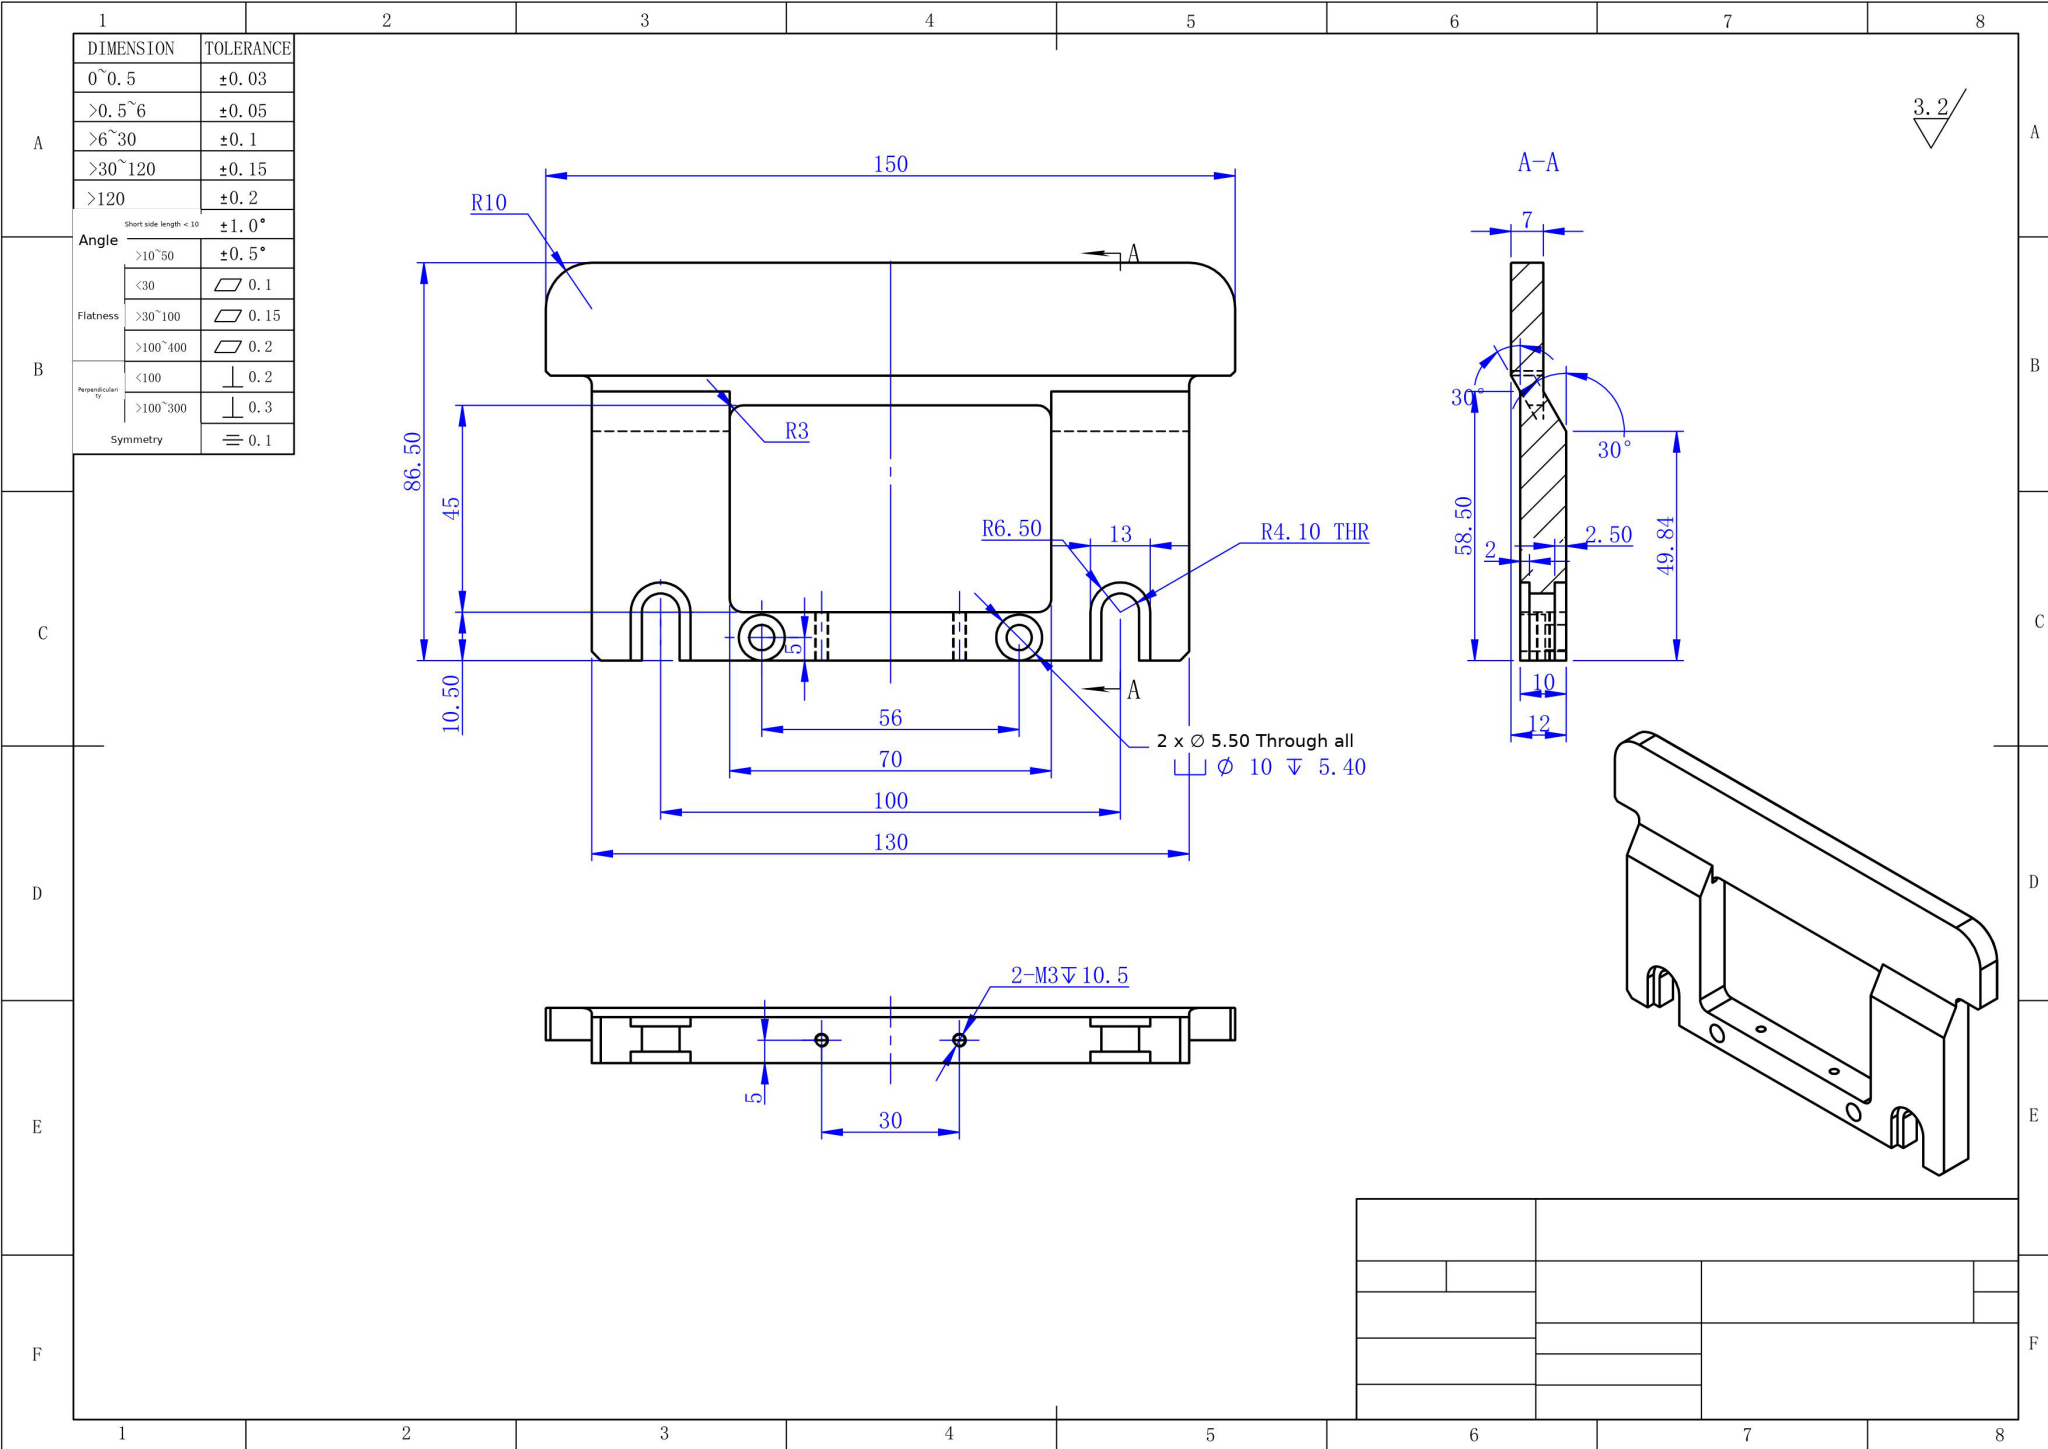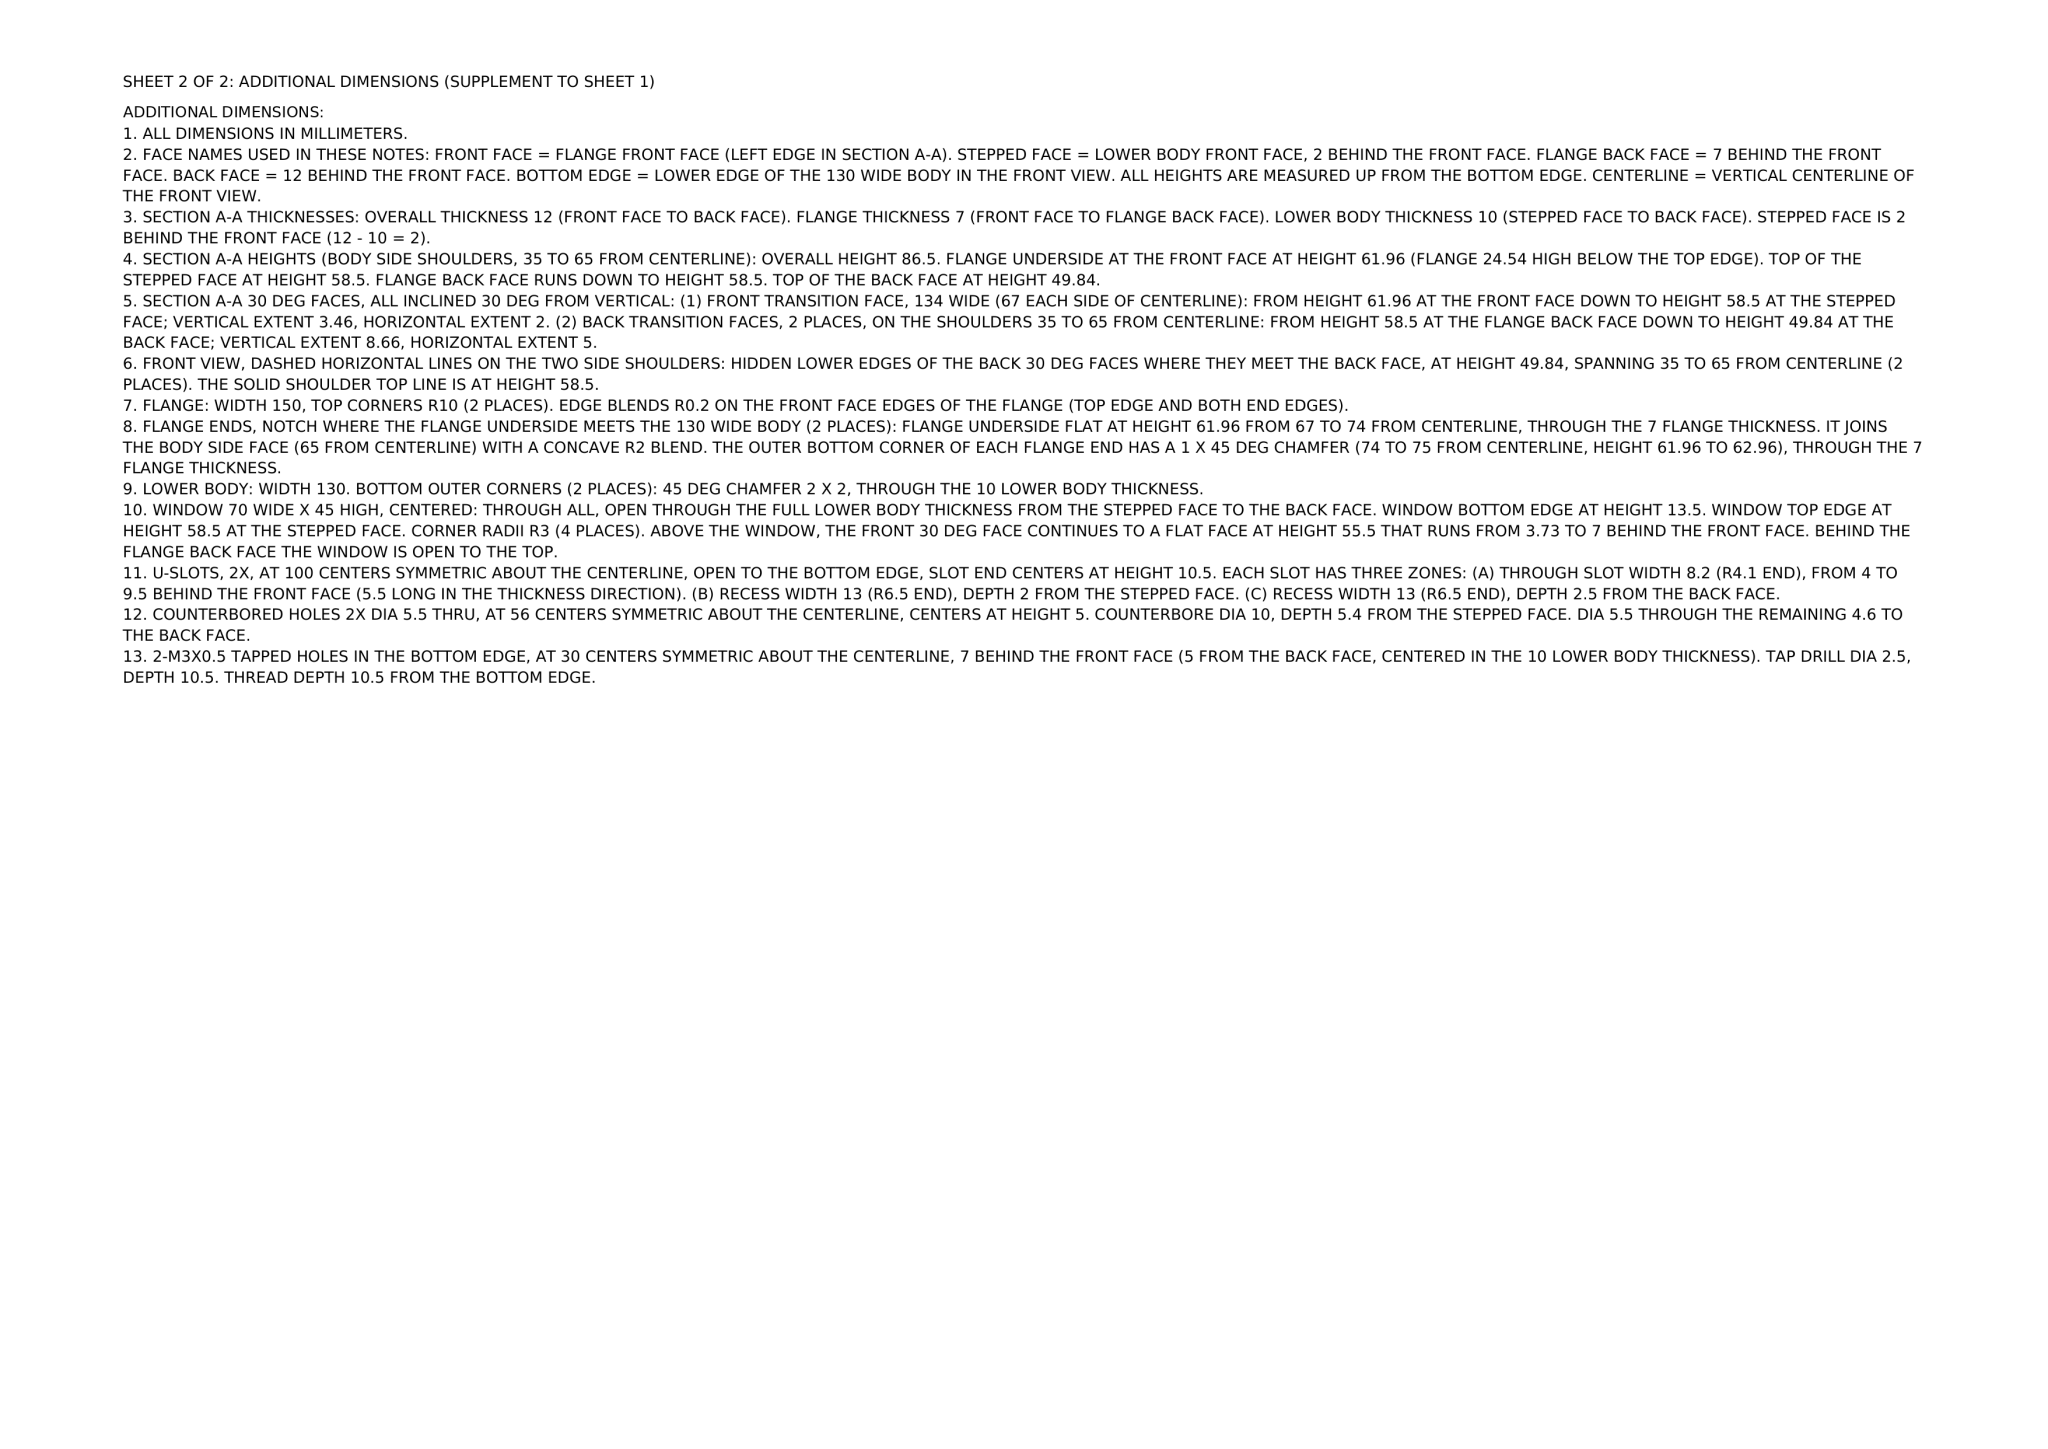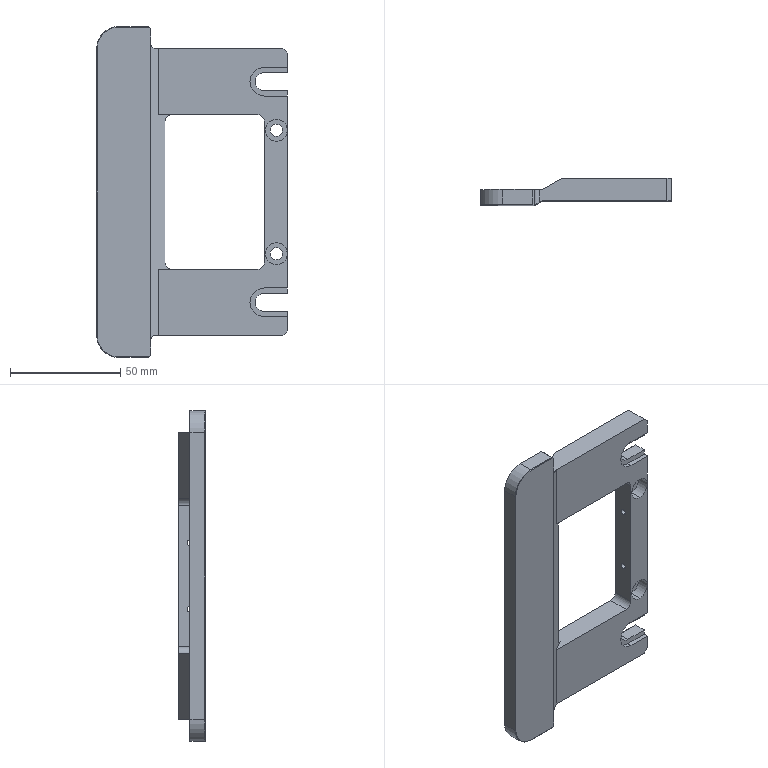Part | NX | mm | 1 solid | 76 faces | box 86.5 x 12 x 150 mm | volume 65963 mm3 | plane 43 | cylinder 31 | torus 2 | commonest cylinder face diameters 13 x6 2.5 x4 9.999 x4 5.5 x4 6 x4 0.4 x3 8.2 x2 20 x2